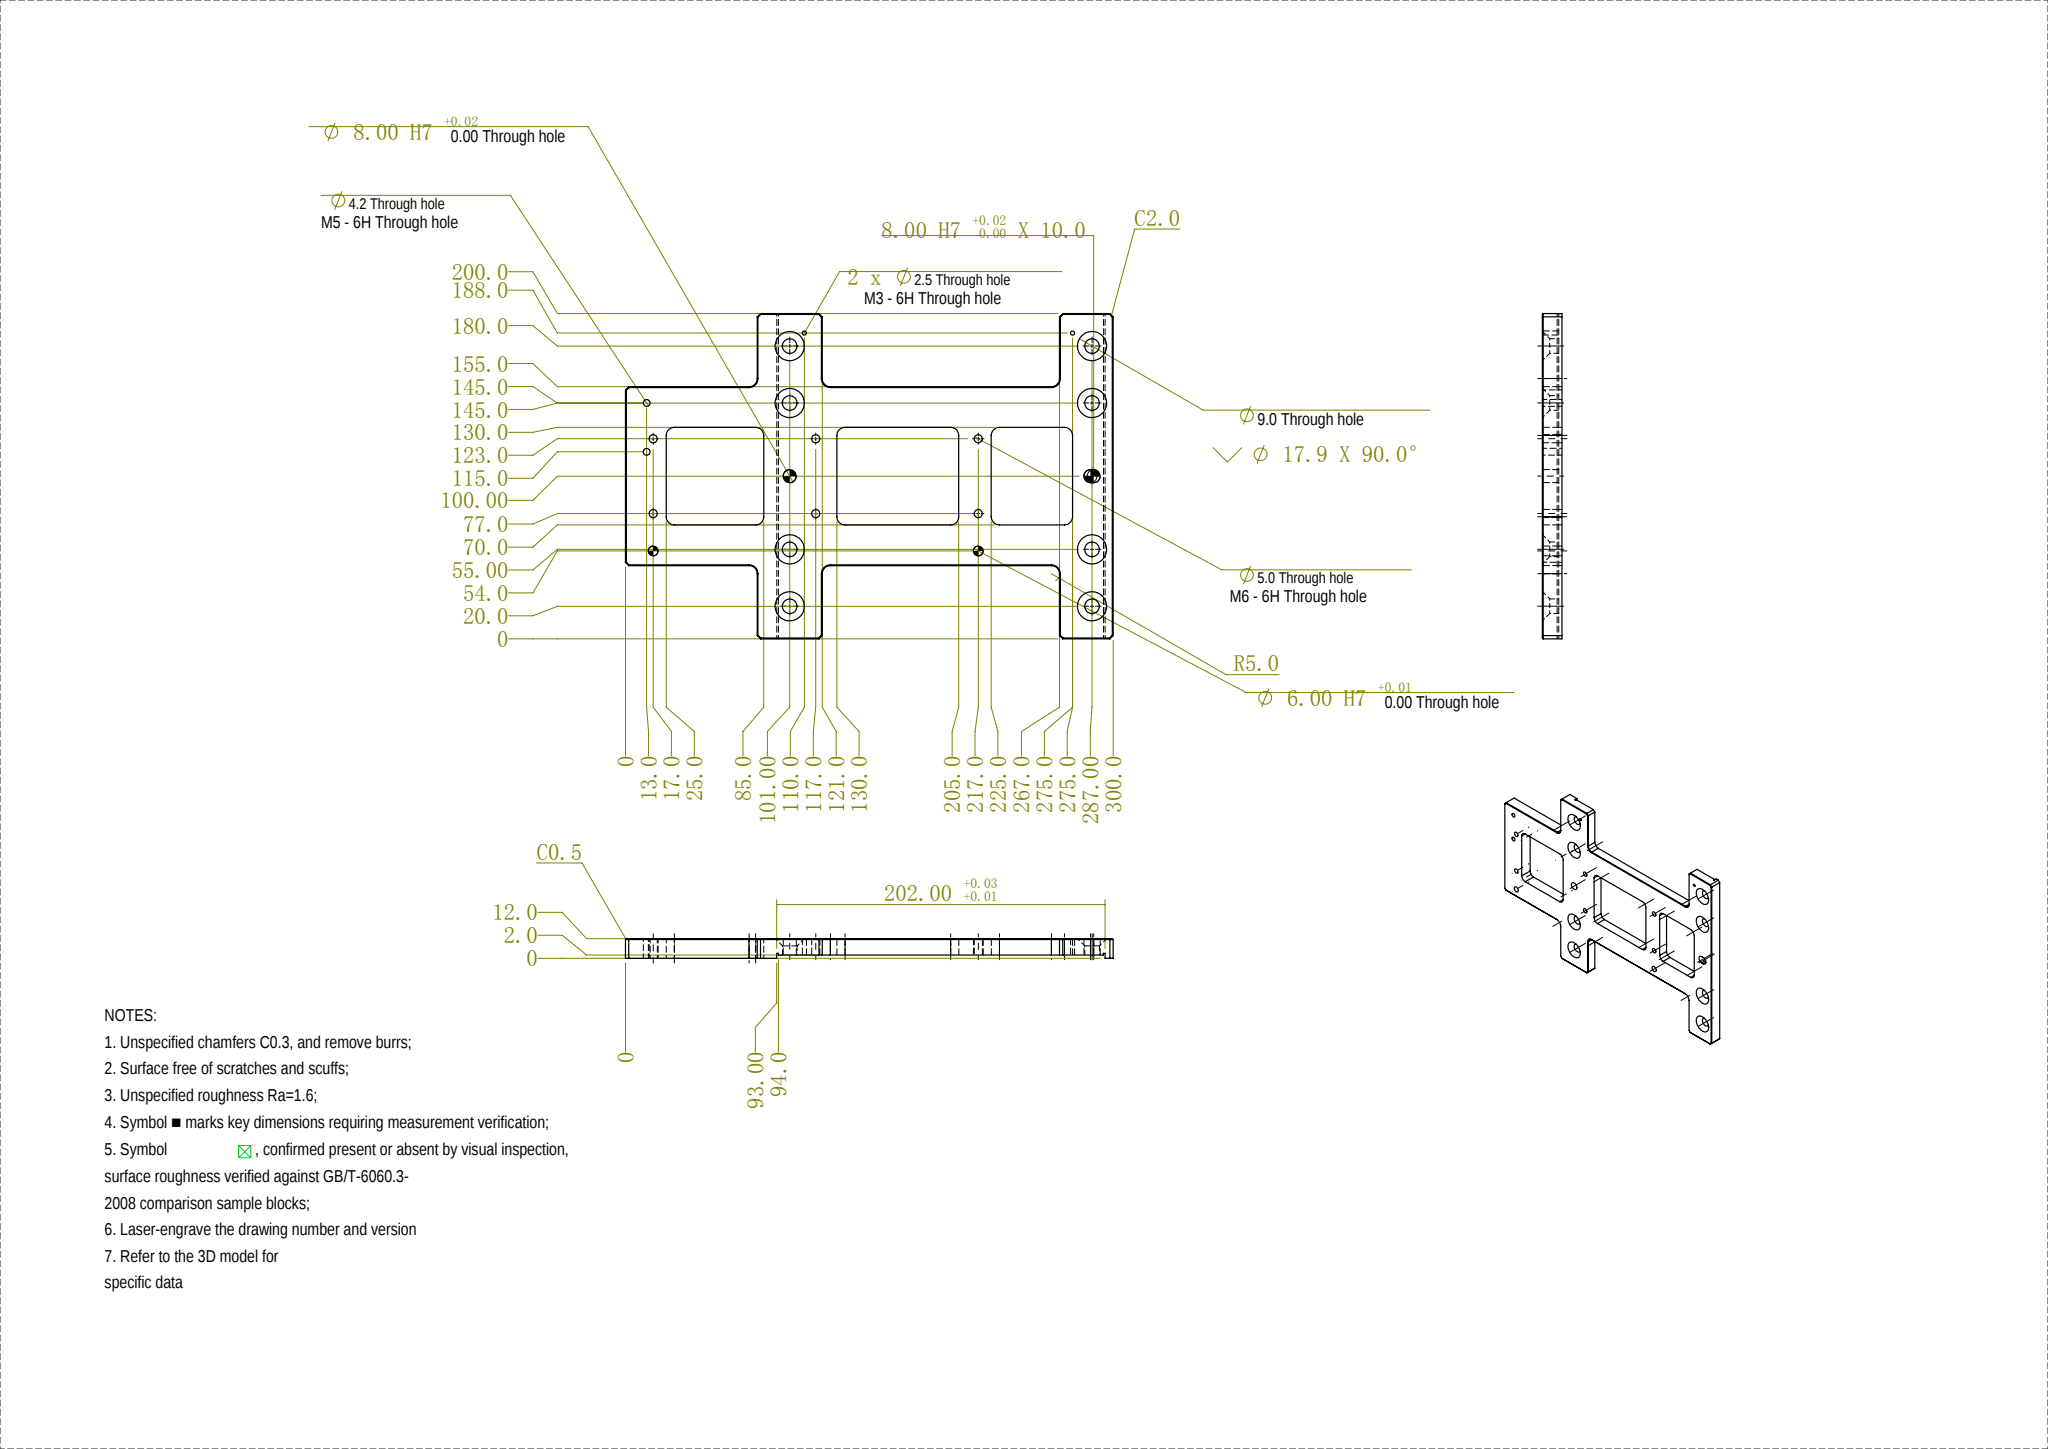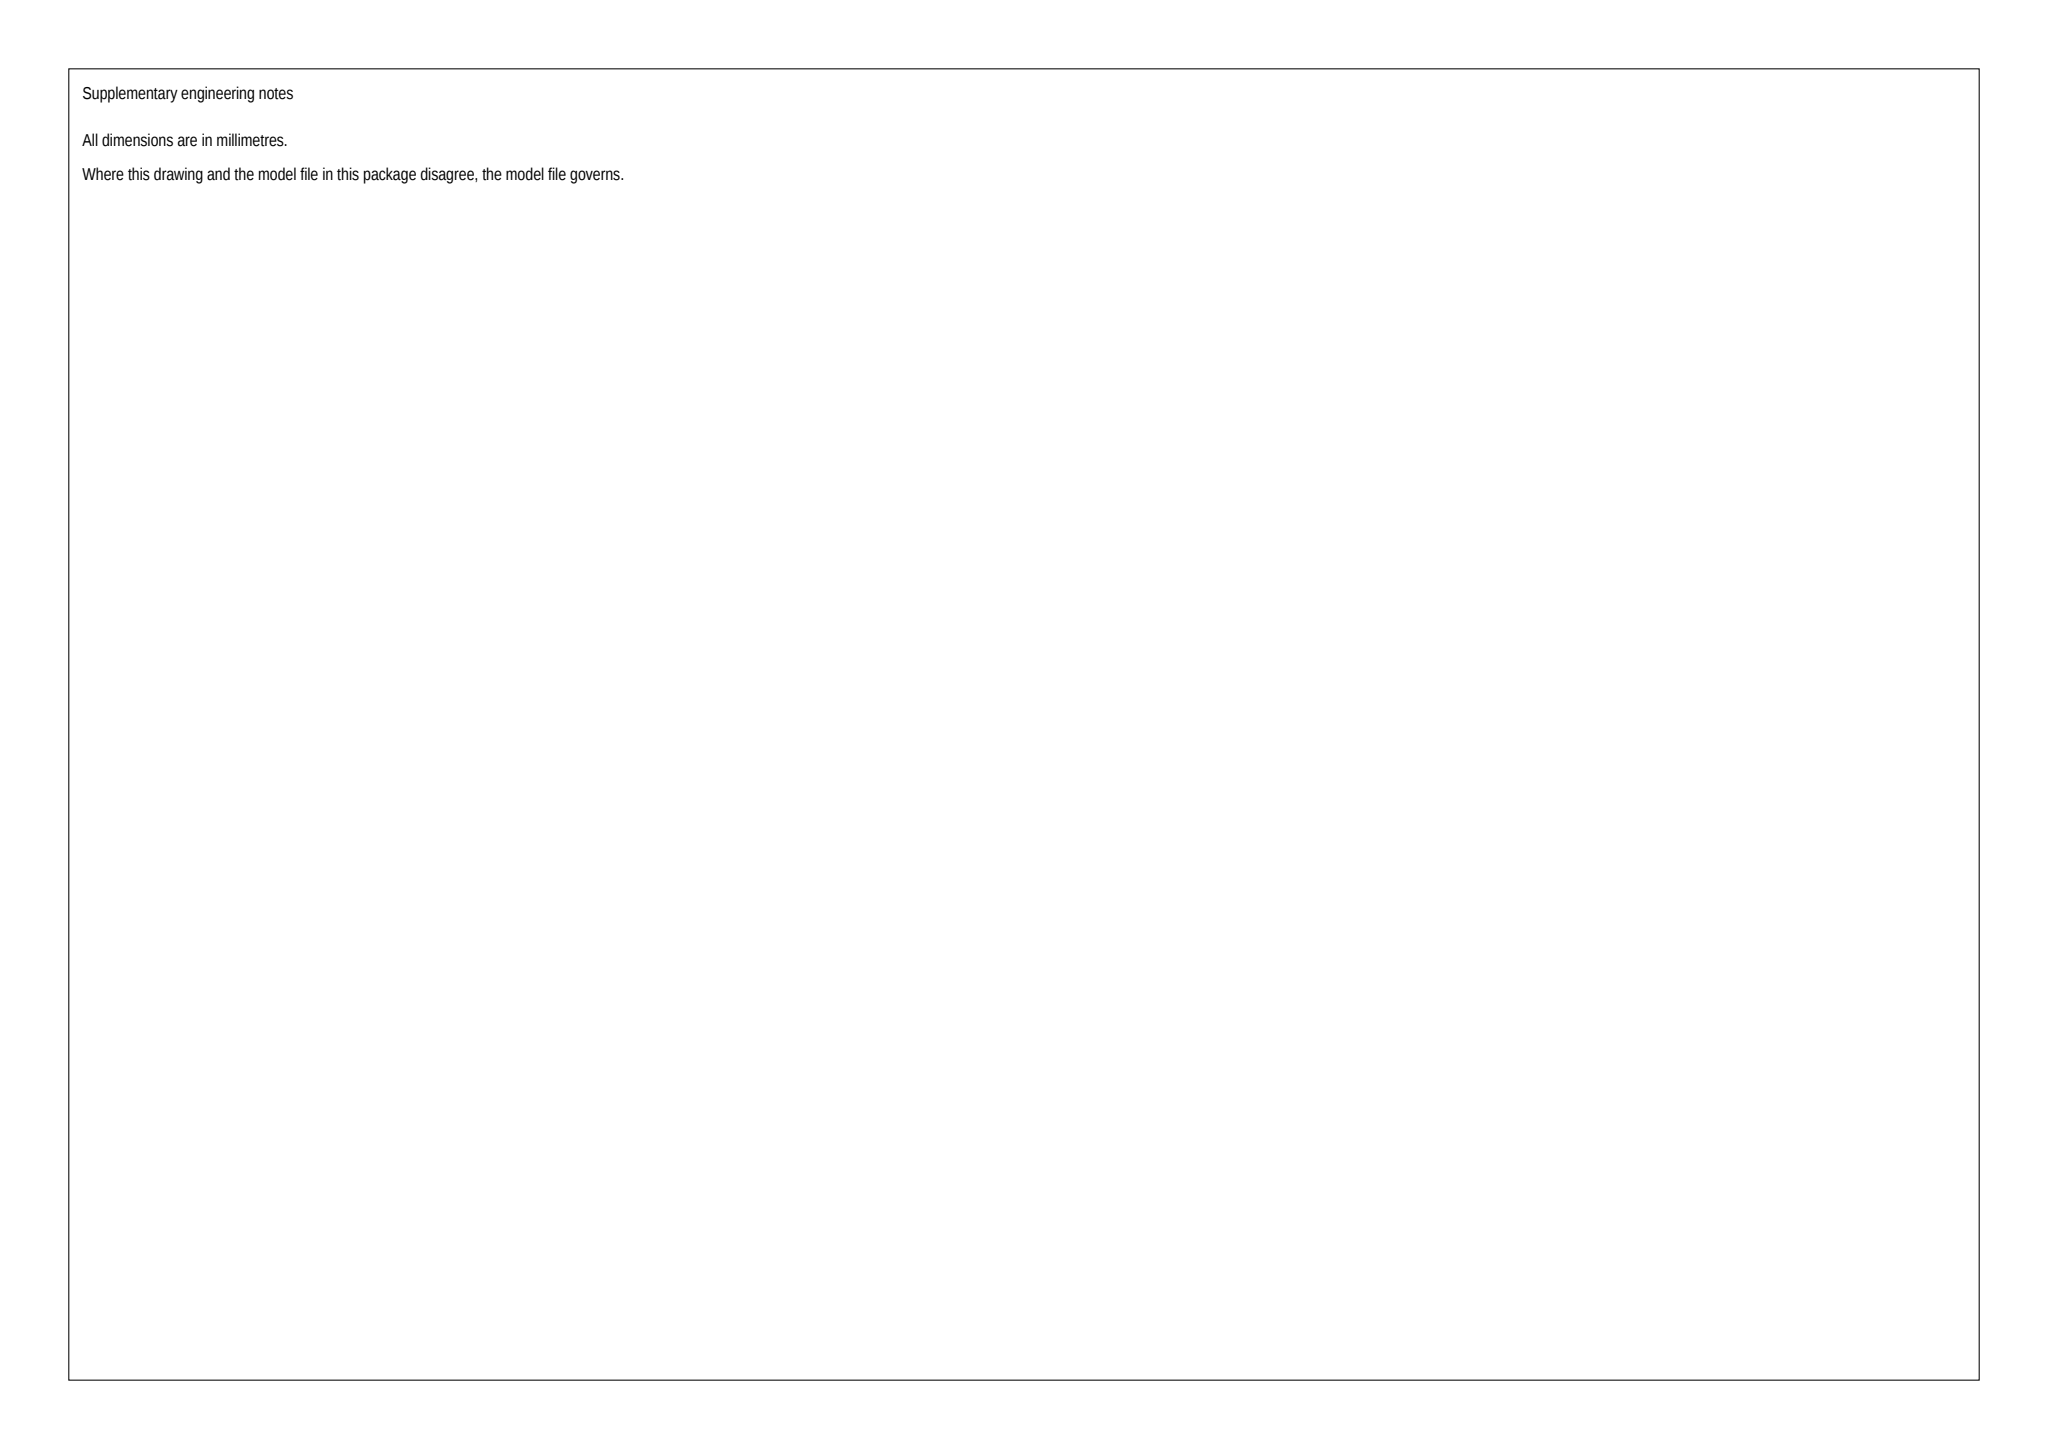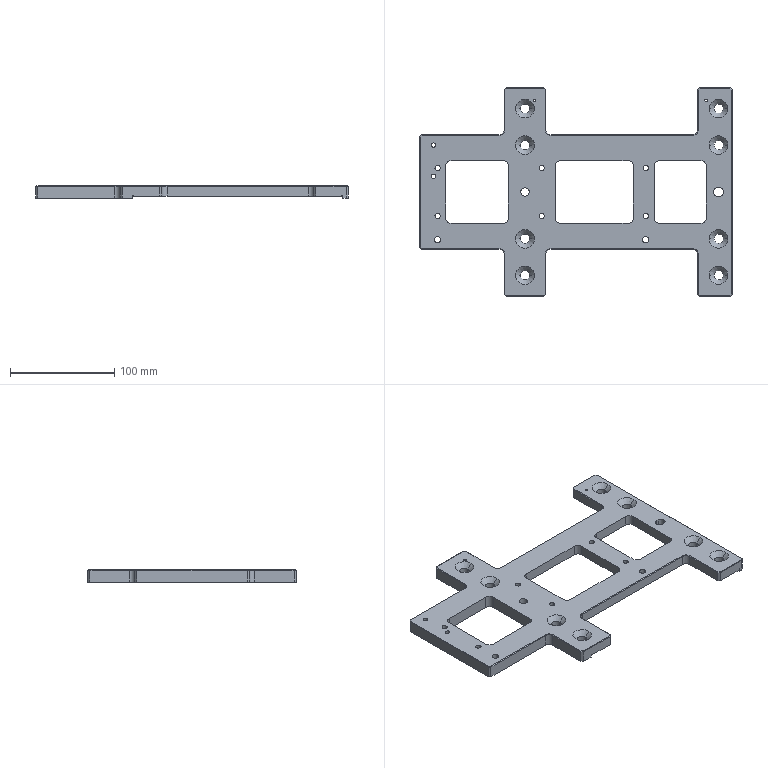Part | SolidWorks | mm | 1 solid | 161 faces | box 300 x 200 x 12 mm | volume 290825 mm3 | plane 76 | cylinder 63 | cone 22 | commonest cylinder face diameters 10 x18 9 x16 5 x12 8 x5 2.5 x4 4.2 x4 6 x4
build123d program:
from build123d import *

# Parameters (mm, degrees)
SKETCH1_W                                            = 300
SKETCH1_H                                            = 200
BOSS_EXTRUDE1_DEPTH                                  = 6
SKETCH3_W                                            = 202
SKETCH3_H                                            = 200
CUT_EXTRUDE1_DEPTH                                   = 2
TAPERED_COUNTERSUNK_HOLE_1_FOR_M8_HEXAGO_D           = 9
TAPERED_COUNTERSUNK_HOLE_1_FOR_M8_HEXAGO_CSINK_D     = 17.92
TAPERED_COUNTERSUNK_HOLE_1_FOR_M8_HEXAGO_CSINK_ANGLE = 90
SIZE_MM_DOWEL_PIN_HOLE_1_D                           = 8
CUT_EXTRUDE2_DEPTH                                   = 181.677
CUT_EXTRUDE3_DEPTH                                   = 181.677
M6_TAPPED_HOLE1_D                                    = 5
SIZE_MM_DOWEL_PIN_HOLE_2_D                           = 6
CUT_EXTRUDE4_DEPTH                                   = 181.677
CHAMFER1_SIZE                                        = 2
SKETCH15_W                                           = 1
SKETCH15_H                                           = 1
CUT_EXTRUDE5_DEPTH                                   = 296
CHAMFER2_SIZE                                        = 0.5
M5_TAPPED_HOLE1_D                                    = 4.2
M3_TAPPED_HOLE1_D                                    = 2.5


with BuildPart() as part:
    # Sketch1 → Boss-Extrude1 (new, symmetric)
    with BuildSketch(Plane.XY):
        Rectangle(SKETCH1_W, SKETCH1_H)
    extrude(amount=BOSS_EXTRUDE1_DEPTH, both=True)

    # Sketch3 → Cut-Extrude1 (cut)
    with BuildSketch(Plane(origin=(0, 0, -6), x_dir=(-1, 0, 0), z_dir=(0, 0, -1))):
        with Locations((-44, 0)):
            Rectangle(SKETCH3_W, SKETCH3_H)
    extrude(amount=-CUT_EXTRUDE1_DEPTH, mode=Mode.SUBTRACT)

    # Tapered Countersunk Hole 1 for M8 Hexago (through all)
    with Locations(Plane.XY.offset(6)):
        with Locations((137, -80), (137, 80), (137, 45), (137, -45), (-49, -45), (-49, 45), (-49, 80), (-49, -80)):
            CounterSinkHole(TAPERED_COUNTERSUNK_HOLE_1_FOR_M8_HEXAGO_D / 2, TAPERED_COUNTERSUNK_HOLE_1_FOR_M8_HEXAGO_CSINK_D / 2, counter_sink_angle=TAPERED_COUNTERSUNK_HOLE_1_FOR_M8_HEXAGO_CSINK_ANGLE)

    # Size mm Dowel Pin Hole 1 (through all)
    with Locations(Plane.XY.offset(6)):
        with Locations((137, 0), (-49, 0)):
            Hole(SIZE_MM_DOWEL_PIN_HOLE_1_D / 2)

    # Sketch8 → Cut-Extrude2 (cut, through all)
    with BuildSketch(Plane.XY.offset(6)):
        with BuildLine():
            Line((136, 4), (138, 4))
            ThreePointArc((138, 4), (142, 0), (138, -4))
            Line((138, -4), (136, -4))
            ThreePointArc((136, -4), (132, 0), (136, 4))
        make_face()
    extrude(amount=-CUT_EXTRUDE2_DEPTH, mode=Mode.SUBTRACT)

    # Sketch9 → Cut-Extrude3 (cut, through all)
    with BuildSketch(Plane(origin=(0, 0, -6), x_dir=(-1, 0, 0), z_dir=(0, 0, -1))):
        with BuildLine():
            Line((150, 100), (69, 100))
            Line((69, 100), (69, 60))
            ThreePointArc((69, 60), (70.464, 56.464), (74, 55))
            Line((74, 55), (150, 55))
            Line((150, 55), (150, 100))
        make_face()
        with BuildLine():
            Line((150, -100), (69, -100))
            Line((69, -100), (69, -60))
            ThreePointArc((69, -60), (70.464, -56.464), (74, -55))
            Line((74, -55), (150, -55))
            Line((150, -55), (150, -100))
        make_face()
        with BuildLine():
            Line((29, 100), (-117, 100))
            Line((-117, 100), (-117, 60))
            ThreePointArc((-117, 60), (-115.536, 56.464), (-112, 55))
            Line((-112, 55), (24, 55))
            ThreePointArc((24, 55), (27.536, 56.464), (29, 60))
            Line((29, 60), (29, 100))
        make_face()
        with BuildLine():
            Line((29, -100), (-117, -100))
            Line((-117, -100), (-117, -60))
            ThreePointArc((-117, -60), (-115.536, -56.464), (-112, -55))
            Line((-112, -55), (24, -55))
            ThreePointArc((24, -55), (27.536, -56.464), (29, -60))
            Line((29, -60), (29, -100))
        make_face()
    extrude(amount=-CUT_EXTRUDE3_DEPTH, mode=Mode.SUBTRACT)

    # M6 Tapped Hole1 (through all)
    with Locations(Plane.XY.offset(6)):
        with Locations((-133, -23), (-133, 23), (-33, -23), (-33, 23), (67, -23), (67, 23)):
            Hole(M6_TAPPED_HOLE1_D / 2)

    # Size mm Dowel Pin Hole 2 (through all)
    with Locations(Plane.XY.offset(6)):
        with Locations((-133, -46), (67, -46)):
            Hole(SIZE_MM_DOWEL_PIN_HOLE_2_D / 2)

    # Sketch14 → Cut-Extrude4 (cut, through all)
    with BuildSketch(Plane.XY.offset(6)):
        with BuildLine():
            Line((-120, -30), (-70, -30))
            ThreePointArc((-70, -30), (-66.464, -28.536), (-65, -25))
            Line((-65, -25), (-65, 25))
            ThreePointArc((-65, 25), (-66.464, 28.536), (-70, 30))
            Line((-70, 30), (-120, 30))
            ThreePointArc((-120, 30), (-123.536, 28.536), (-125, 25))
            Line((-125, 25), (-125, -25))
            ThreePointArc((-125, -25), (-123.536, -28.536), (-120, -30))
        make_face()
        with BuildLine():
            Line((-15, -30), (50, -30))
            ThreePointArc((50, -30), (53.536, -28.536), (55, -25))
            Line((55, -25), (55, 25))
            ThreePointArc((55, 25), (53.536, 28.536), (50, 30))
            Line((50, 30), (-15, 30))
            ThreePointArc((-15, 30), (-18.536, 28.536), (-20, 25))
            Line((-20, 25), (-20, -25))
            ThreePointArc((-20, -25), (-18.536, -28.536), (-15, -30))
        make_face()
        with BuildLine():
            Line((80, -30), (120, -30))
            ThreePointArc((120, -30), (123.536, -28.536), (125, -25))
            Line((125, -25), (125, 25))
            ThreePointArc((125, 25), (123.536, 28.536), (120, 30))
            Line((120, 30), (80, 30))
            ThreePointArc((80, 30), (76.464, 28.536), (75, 25))
            Line((75, 25), (75, -25))
            ThreePointArc((75, -25), (76.464, -28.536), (80, -30))
        make_face()
    extrude(amount=-CUT_EXTRUDE4_DEPTH, mode=Mode.SUBTRACT)

    # Chamfer1
    chamfer1_edges = [part.edges().sort_by_distance(p)[0] for p in [
        (-150, -55, 0),
        (-69, -100, 0),
        (-29, 100, 1),
        (117, 100, 1),
        (-29, -100, 1),
        (117, -100, 1),
        (-150, 55, 0),
        (-69, 100, 0),
        (150, -100, 0),
        (150, 100, 0),
    ]]
    chamfer(chamfer1_edges, length=CHAMFER1_SIZE)

    # Sketch15 → Cut-Extrude5 (cut)
    with BuildSketch(Plane.XZ.offset(100)):
        with Locations((-56.5, -3.5)):
            Rectangle(SKETCH15_W, SKETCH15_H)
        with Locations((144.5, -3.5)):
            Rectangle(SKETCH15_W, SKETCH15_H)
    extrude(amount=-CUT_EXTRUDE5_DEPTH, mode=Mode.SUBTRACT)

    # Chamfer2
    chamfer2_edges = [part.edges().sort_by_distance(p)[0] for p in [
        (-69, -79, 6),
        (-70.464, -56.464, 6),
        (-29, 79, 6),
        (-27.536, 56.464, 6),
        (44, 55, 6),
        (115.536, 56.464, 6),
        (117, -79, 6),
        (115.536, -56.464, 6),
        (44, -55, 6),
        (-27.536, -56.464, 6),
        (-111, 55, 6),
        (-70.464, 56.464, 6),
        (117, 79, 6),
        (133.5, 100, 6),
        (-49, -100, 6),
        (-29, -79, 6),
        (133.5, -100, 6),
        (150, 0, 6),
        (-49, 100, 6),
        (-69, 79, 6),
        (-150, 0, 6),
        (-111, -55, 6),
        (-149, -54, 6),
        (-149, 54, 6),
        (-68, 99, 6),
        (-30, 99, 6),
        (149, 99, 6),
        (149, -99, 6),
        (118, -99, 6),
        (-30, -99, 6),
        (-68, -99, 6),
        (118, 99, 6),
    ]]
    chamfer(chamfer2_edges, length=CHAMFER2_SIZE)

    # M5 Tapped Hole1 (through all)
    with Locations(Plane(origin=(0, 0, -6), x_dir=(-1, 0, 0), z_dir=(0, 0, -1))):
        with Locations((137, 45), (137, 15)):
            Hole(M5_TAPPED_HOLE1_D / 2)

    # M3 Tapped Hole1 (through all)
    with Locations(Plane.XY.offset(6)):
        with Locations((-40, 119), (-40, 88), (125, 119), (125, 88)):
            Hole(M3_TAPPED_HOLE1_D / 2)


solid = part.part